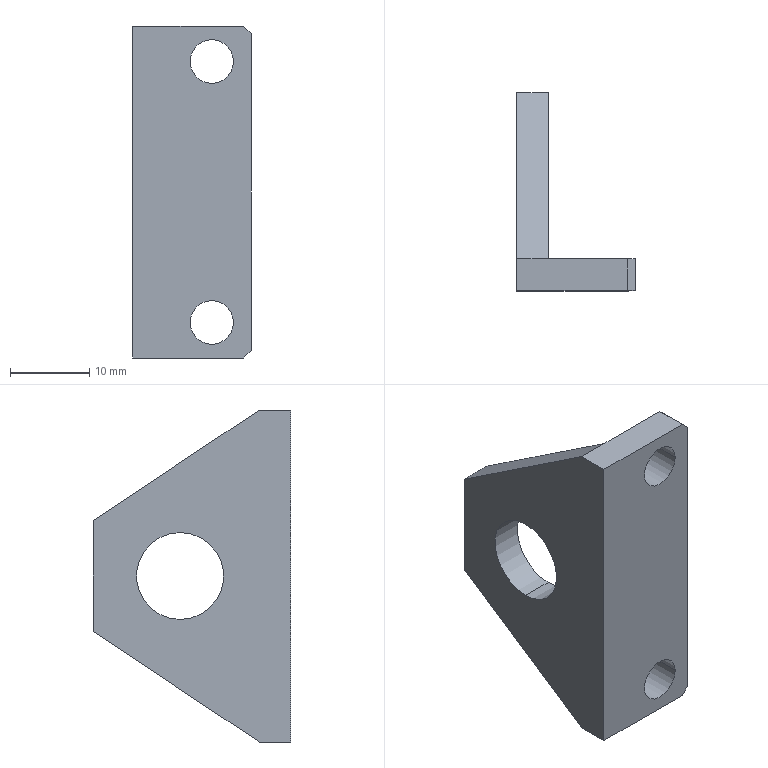Component | SolidWorks | 60100040019CylinderSupport-1 | 1 solid | 18 faces | box 15 x 25 x 42 mm | volume 4298 mm3 | plane 12 | cylinder 6 | commonest cylinder face diameters 5.5 x4 11 x2 | material Q235-A
build123d program:
from build123d import *

# Parameters (mm, degrees)
BOSS_EXTRUDE1_DEPTH = 4
SKETCH2_W           = 42
SKETCH2_H           = 4
BOSS_EXTRUDE2_DEPTH = 15
SKETCH3_R           = 5.5
CUT_EXTRUDE1_DEPTH  = 35.453
SKETCH4_R           = 2.75
CUT_EXTRUDE2_DEPTH  = 34.272
CHAMFER1_SIZE       = 1


with BuildPart() as part:
    # Sketch1 → Boss-Extrude1 (new body)
    with BuildSketch(Plane.XY):
        Polygon((-21, 0), (21, 0), (21, 4), (7, 25), (-7, 25), (-21, 4), align=None)
    extrude(amount=BOSS_EXTRUDE1_DEPTH)

    # Sketch2 → Boss-Extrude2 (add)
    with BuildSketch(Plane.XY):
        with Locations((0, 2)):
            Rectangle(SKETCH2_W, SKETCH2_H)
    extrude(amount=BOSS_EXTRUDE2_DEPTH)

    # Sketch3 → Cut-Extrude1 (cut, through all)
    with BuildSketch(Plane.XY.offset(4)):
        with Locations((0, 14)):
            Circle(SKETCH3_R)
    extrude(amount=-CUT_EXTRUDE1_DEPTH, mode=Mode.SUBTRACT)

    # Sketch4 → Cut-Extrude2 (cut, through all)
    with BuildSketch(Plane(origin=(0, 4, 0), x_dir=(1, 0, 0), z_dir=(0, 1, 0))):
        with Locations(Location((16.5, -10, 0), (0, 0, 270))):
            Circle(SKETCH4_R)
        with Locations(Location((-16.5, -10, 0), (0, 0, 270))):
            Circle(SKETCH4_R)
    extrude(amount=-CUT_EXTRUDE2_DEPTH, mode=Mode.SUBTRACT)

    # Chamfer1
    chamfer1_edges = [part.edges().sort_by_distance(p)[0] for p in [
        (-21, 2, 15),
        (21, 2, 15),
    ]]
    chamfer(chamfer1_edges, length=CHAMFER1_SIZE)


solid = part.part

# Placed as in the assembly
solid = solid.moved(Location((37.27, 8.768, 80.829), (0, 90, 0)))
STEP:
#1=COLOUR_RGB('',0.7922,0.8196,0.9333);
#2=FILL_AREA_STYLE_COLOUR('',#1);
#3=FILL_AREA_STYLE('',(#2));
#4=SURFACE_STYLE_FILL_AREA(#3);
#5=SURFACE_SIDE_STYLE('',(#4));
#6=SURFACE_STYLE_USAGE(.BOTH.,#5);
#7=PRESENTATION_STYLE_ASSIGNMENT((#6));
#8=CARTESIAN_POINT('',(1.753,0.3452,3.832));
#9=VERTEX_POINT('',#8);
#10=CARTESIAN_POINT('',(1.969,0.3452,3.832));
#11=VERTEX_POINT('',#10);
#12=CARTESIAN_POINT('',(1.861,0.3452,3.832));
#13=DIRECTION('',(0.,1.,0.));
#14=DIRECTION('',(1.,0.,0.));
#15=AXIS2_PLACEMENT_3D('',#12,#13,#14);
#16=CIRCLE('',#15,0.1083);
#17=EDGE_CURVE('',#9,#11,#16,.T.);
#18=ORIENTED_EDGE('',*,*,#17,.F.);
#19=CARTESIAN_POINT('',(1.753,0.5027,3.832));
#20=VERTEX_POINT('',#19);
#21=CARTESIAN_POINT('',(1.753,0.3452,3.832));
#22=DIRECTION('',(0.,1.,0.));
#23=VECTOR('',#22,39.37);
#24=LINE('',#21,#23);
#25=EDGE_CURVE('',#9,#20,#24,.T.);
#26=ORIENTED_EDGE('',*,*,#25,.T.);
#27=CARTESIAN_POINT('',(1.969,0.5027,3.832));
#28=VERTEX_POINT('',#27);
#29=CARTESIAN_POINT('',(1.861,0.5027,3.832));
#30=DIRECTION('',(0.,1.,0.));
#31=DIRECTION('',(1.,0.,0.));
#32=AXIS2_PLACEMENT_3D('',#29,#30,#31);
#33=CIRCLE('',#32,0.1083);
#34=EDGE_CURVE('',#20,#28,#33,.T.);
#35=ORIENTED_EDGE('',*,*,#34,.T.);
#36=CARTESIAN_POINT('',(1.969,0.3452,3.832));
#37=DIRECTION('',(0.,1.,0.));
#38=VECTOR('',#37,39.37);
#39=LINE('',#36,#38);
#40=EDGE_CURVE('',#11,#28,#39,.T.);
#41=ORIENTED_EDGE('',*,*,#40,.F.);
#42=EDGE_LOOP('',(#18,#26,#35,#41));
#43=FACE_OUTER_BOUND('',#42,.T.);
#44=CARTESIAN_POINT('',(1.861,0.3452,3.832));
#45=DIRECTION('',(0.,1.,0.));
#46=DIRECTION('',(1.,0.,0.));
#47=AXIS2_PLACEMENT_3D('',#44,#45,#46);
#48=CYLINDRICAL_SURFACE('',#47,0.1083);
#49=ADVANCED_FACE('',(#43),#48,.F.);
#50=CARTESIAN_POINT('',(1.753,0.3452,2.533));
#51=VERTEX_POINT('',#50);
#52=CARTESIAN_POINT('',(1.969,0.3452,2.533));
#53=VERTEX_POINT('',#52);
#54=CARTESIAN_POINT('',(1.861,0.3452,2.533));
#55=DIRECTION('',(0.,1.,0.));
#56=DIRECTION('',(1.,0.,0.));
#57=AXIS2_PLACEMENT_3D('',#54,#55,#56);
#58=CIRCLE('',#57,0.1083);
#59=EDGE_CURVE('',#51,#53,#58,.T.);
#60=ORIENTED_EDGE('',*,*,#59,.F.);
#61=CARTESIAN_POINT('',(1.753,0.5027,2.533));
#62=VERTEX_POINT('',#61);
#63=CARTESIAN_POINT('',(1.753,0.3452,2.533));
#64=DIRECTION('',(0.,1.,0.));
#65=VECTOR('',#64,39.37);
#66=LINE('',#63,#65);
#67=EDGE_CURVE('',#51,#62,#66,.T.);
#68=ORIENTED_EDGE('',*,*,#67,.T.);
#69=CARTESIAN_POINT('',(1.969,0.5027,2.533));
#70=VERTEX_POINT('',#69);
#71=CARTESIAN_POINT('',(1.861,0.5027,2.533));
#72=DIRECTION('',(0.,1.,0.));
#73=DIRECTION('',(1.,0.,0.));
#74=AXIS2_PLACEMENT_3D('',#71,#72,#73);
#75=CIRCLE('',#74,0.1083);
#76=EDGE_CURVE('',#62,#70,#75,.T.);
#77=ORIENTED_EDGE('',*,*,#76,.T.);
#78=CARTESIAN_POINT('',(1.969,0.3452,2.533));
#79=DIRECTION('',(0.,1.,0.));
#80=VECTOR('',#79,39.37);
#81=LINE('',#78,#80);
#82=EDGE_CURVE('',#53,#70,#81,.T.);
#83=ORIENTED_EDGE('',*,*,#82,.F.);
#84=EDGE_LOOP('',(#60,#68,#77,#83));
#85=FACE_OUTER_BOUND('',#84,.T.);
#86=CARTESIAN_POINT('',(1.861,0.3452,2.533));
#87=DIRECTION('',(0.,1.,0.));
#88=DIRECTION('',(1.,0.,0.));
#89=AXIS2_PLACEMENT_3D('',#86,#87,#88);
#90=CYLINDRICAL_SURFACE('',#89,0.1083);
#91=ADVANCED_FACE('',(#85),#90,.F.);
#92=CARTESIAN_POINT('',(1.467,0.8964,3.399));
#93=VERTEX_POINT('',#92);
#94=CARTESIAN_POINT('',(1.467,0.8964,2.966));
#95=VERTEX_POINT('',#94);
#96=CARTESIAN_POINT('',(1.467,0.8964,3.182));
#97=DIRECTION('',(1.,0.,0.));
#98=DIRECTION('',(0.,0.,-1.));
#99=AXIS2_PLACEMENT_3D('',#96,#97,#98);
#100=CIRCLE('',#99,0.2165);
#101=EDGE_CURVE('',#93,#95,#100,.T.);
#102=ORIENTED_EDGE('',*,*,#101,.F.);
#103=CARTESIAN_POINT('',(1.625,0.8964,3.399));
#104=VERTEX_POINT('',#103);
#105=CARTESIAN_POINT('',(1.467,0.8964,3.399));
#106=DIRECTION('',(1.,0.,0.));
#107=VECTOR('',#106,39.37);
#108=LINE('',#105,#107);
#109=EDGE_CURVE('',#93,#104,#108,.T.);
#110=ORIENTED_EDGE('',*,*,#109,.T.);
#111=CARTESIAN_POINT('',(1.625,0.8964,2.966));
#112=VERTEX_POINT('',#111);
#113=CARTESIAN_POINT('',(1.625,0.8964,3.182));
#114=DIRECTION('',(1.,0.,0.));
#115=DIRECTION('',(0.,0.,-1.));
#116=AXIS2_PLACEMENT_3D('',#113,#114,#115);
#117=CIRCLE('',#116,0.2165);
#118=EDGE_CURVE('',#104,#112,#117,.T.);
#119=ORIENTED_EDGE('',*,*,#118,.T.);
#120=CARTESIAN_POINT('',(1.467,0.8964,2.966));
#121=DIRECTION('',(1.,0.,0.));
#122=VECTOR('',#121,39.37);
#123=LINE('',#120,#122);
#124=EDGE_CURVE('',#95,#112,#123,.T.);
#125=ORIENTED_EDGE('',*,*,#124,.F.);
#126=EDGE_LOOP('',(#102,#110,#119,#125));
#127=FACE_OUTER_BOUND('',#126,.T.);
#128=CARTESIAN_POINT('',(1.467,0.8964,3.182));
#129=DIRECTION('',(1.,0.,0.));
#130=DIRECTION('',(0.,0.,-1.));
#131=AXIS2_PLACEMENT_3D('',#128,#129,#130);
#132=CYLINDRICAL_SURFACE('',#131,0.2165);
#133=ADVANCED_FACE('',(#127),#132,.F.);
#134=CARTESIAN_POINT('',(1.625,0.8964,3.182));
#135=DIRECTION('',(1.,0.,0.));
#136=DIRECTION('',(0.,0.,-1.));
#137=AXIS2_PLACEMENT_3D('',#134,#135,#136);
#138=CIRCLE('',#137,0.2165);
#139=EDGE_CURVE('',#112,#104,#138,.T.);
#140=ORIENTED_EDGE('',*,*,#139,.F.);
#141=ORIENTED_EDGE('',*,*,#118,.F.);
#142=EDGE_LOOP('',(#140,#141));
#143=FACE_BOUND('',#142,.T.);
#144=CARTESIAN_POINT('',(1.625,1.329,3.458));
#145=VERTEX_POINT('',#144);
#146=CARTESIAN_POINT('',(1.625,0.5027,4.009));
#147=VERTEX_POINT('',#146);
#148=CARTESIAN_POINT('',(1.625,1.329,3.458));
#149=DIRECTION('',(0.,-0.8321,0.5547));
#150=VECTOR('',#149,39.37);
#151=LINE('',#148,#150);
#152=EDGE_CURVE('',#145,#147,#151,.T.);
#153=ORIENTED_EDGE('',*,*,#152,.T.);
#154=CARTESIAN_POINT('',(1.625,0.5027,2.355));
#155=VERTEX_POINT('',#154);
#156=CARTESIAN_POINT('',(1.625,0.5027,4.009));
#157=DIRECTION('',(0.,0.,-1.));
#158=VECTOR('',#157,39.37);
#159=LINE('',#156,#158);
#160=EDGE_CURVE('',#147,#155,#159,.T.);
#161=ORIENTED_EDGE('',*,*,#160,.T.);
#162=CARTESIAN_POINT('',(1.625,1.329,2.907));
#163=VERTEX_POINT('',#162);
#164=CARTESIAN_POINT('',(1.625,1.329,2.907));
#165=DIRECTION('',(0.,0.8321,0.5547));
#166=VECTOR('',#165,39.37);
#167=LINE('',#164,#166);
#168=EDGE_CURVE('',#155,#163,#167,.T.);
#169=ORIENTED_EDGE('',*,*,#168,.T.);
#170=CARTESIAN_POINT('',(1.625,1.329,2.907));
#171=DIRECTION('',(0.,0.,1.));
#172=VECTOR('',#171,39.37);
#173=LINE('',#170,#172);
#174=EDGE_CURVE('',#163,#145,#173,.T.);
#175=ORIENTED_EDGE('',*,*,#174,.T.);
#176=EDGE_LOOP('',(#153,#161,#169,#175));
#177=FACE_OUTER_BOUND('',#176,.T.);
#178=CARTESIAN_POINT('',(1.625,0.3452,4.009));
#179=DIRECTION('',(1.,0.,0.));
#180=DIRECTION('',(0.,0.,-1.));
#181=AXIS2_PLACEMENT_3D('',#178,#179,#180);
#182=PLANE('',#181);
#183=ADVANCED_FACE('',(#143,#177),#182,.T.);
#184=CARTESIAN_POINT('',(2.019,0.3452,4.009));
#185=VERTEX_POINT('',#184);
#186=CARTESIAN_POINT('',(1.467,0.3452,4.009));
#187=VERTEX_POINT('',#186);
#188=CARTESIAN_POINT('',(1.625,0.3452,4.009));
#189=DIRECTION('',(-1.,0.,0.));
#190=VECTOR('',#189,39.37);
#191=LINE('',#188,#190);
#192=EDGE_CURVE('',#185,#187,#191,.T.);
#193=ORIENTED_EDGE('',*,*,#192,.F.);
#194=CARTESIAN_POINT('',(2.019,0.5027,4.009));
#195=VERTEX_POINT('',#194);
#196=CARTESIAN_POINT('',(2.019,0.5027,4.009));
#197=DIRECTION('',(0.,1.,0.));
#198=VECTOR('',#197,39.37);
#199=LINE('',#196,#198);
#200=EDGE_CURVE('',#185,#195,#199,.T.);
#201=ORIENTED_EDGE('',*,*,#200,.T.);
#202=CARTESIAN_POINT('',(2.058,0.5027,4.009));
#203=DIRECTION('',(-1.,0.,0.));
#204=VECTOR('',#203,39.37);
#205=LINE('',#202,#204);
#206=EDGE_CURVE('',#195,#147,#205,.T.);
#207=ORIENTED_EDGE('',*,*,#206,.T.);
#208=CARTESIAN_POINT('',(1.467,0.5027,4.009));
#209=VERTEX_POINT('',#208);
#210=CARTESIAN_POINT('',(1.625,0.5027,4.009));
#211=DIRECTION('',(-1.,0.,0.));
#212=VECTOR('',#211,39.37);
#213=LINE('',#210,#212);
#214=EDGE_CURVE('',#147,#209,#213,.T.);
#215=ORIENTED_EDGE('',*,*,#214,.T.);
#216=CARTESIAN_POINT('',(1.467,0.5027,4.009));
#217=DIRECTION('',(0.,-1.,0.));
#218=VECTOR('',#217,39.37);
#219=LINE('',#216,#218);
#220=EDGE_CURVE('',#209,#187,#219,.T.);
#221=ORIENTED_EDGE('',*,*,#220,.T.);
#222=EDGE_LOOP('',(#193,#201,#207,#215,#221));
#223=FACE_OUTER_BOUND('',#222,.T.);
#224=CARTESIAN_POINT('',(1.625,0.5027,4.009));
#225=DIRECTION('',(0.,0.,-1.));
#226=DIRECTION('',(-1.,0.,0.));
#227=AXIS2_PLACEMENT_3D('',#224,#225,#226);
#228=PLANE('',#227);
#229=ADVANCED_FACE('',(#223),#228,.F.);
#230=CARTESIAN_POINT('',(1.861,0.3452,3.832));
#231=DIRECTION('',(0.,1.,0.));
#232=DIRECTION('',(1.,0.,0.));
#233=AXIS2_PLACEMENT_3D('',#230,#231,#232);
#234=CIRCLE('',#233,0.1083);
#235=EDGE_CURVE('',#11,#9,#234,.T.);
#236=ORIENTED_EDGE('',*,*,#235,.T.);
#237=ORIENTED_EDGE('',*,*,#17,.T.);
#238=EDGE_LOOP('',(#236,#237));
#239=FACE_BOUND('',#238,.T.);
#240=CARTESIAN_POINT('',(1.861,0.3452,2.533));
#241=DIRECTION('',(0.,1.,0.));
#242=DIRECTION('',(1.,0.,0.));
#243=AXIS2_PLACEMENT_3D('',#240,#241,#242);
#244=CIRCLE('',#243,0.1083);
#245=EDGE_CURVE('',#53,#51,#244,.T.);
#246=ORIENTED_EDGE('',*,*,#245,.T.);
#247=ORIENTED_EDGE('',*,*,#59,.T.);
#248=EDGE_LOOP('',(#246,#247));
#249=FACE_BOUND('',#248,.T.);
#250=CARTESIAN_POINT('',(2.019,0.3452,2.355));
#251=VERTEX_POINT('',#250);
#252=CARTESIAN_POINT('',(1.467,0.3452,2.355));
#253=VERTEX_POINT('',#252);
#254=CARTESIAN_POINT('',(1.625,0.3452,2.355));
#255=DIRECTION('',(-1.,0.,0.));
#256=VECTOR('',#255,39.37);
#257=LINE('',#254,#256);
#258=EDGE_CURVE('',#251,#253,#257,.T.);
#259=ORIENTED_EDGE('',*,*,#258,.F.);
#260=CARTESIAN_POINT('',(2.058,0.3452,2.395));
#261=VERTEX_POINT('',#260);
#262=CARTESIAN_POINT('',(2.058,0.3452,2.395));
#263=DIRECTION('',(0.7071,0.,0.7071));
#264=VECTOR('',#263,39.37);
#265=LINE('',#262,#264);
#266=EDGE_CURVE('',#251,#261,#265,.T.);
#267=ORIENTED_EDGE('',*,*,#266,.T.);
#268=CARTESIAN_POINT('',(2.058,0.3452,3.97));
#269=VERTEX_POINT('',#268);
#270=CARTESIAN_POINT('',(2.058,0.3452,4.009));
#271=DIRECTION('',(0.,0.,-1.));
#272=VECTOR('',#271,39.37);
#273=LINE('',#270,#272);
#274=EDGE_CURVE('',#269,#261,#273,.T.);
#275=ORIENTED_EDGE('',*,*,#274,.F.);
#276=CARTESIAN_POINT('',(2.058,0.3452,3.97));
#277=DIRECTION('',(-0.7071,0.,0.7071));
#278=VECTOR('',#277,39.37);
#279=LINE('',#276,#278);
#280=EDGE_CURVE('',#269,#185,#279,.T.);
#281=ORIENTED_EDGE('',*,*,#280,.T.);
#282=ORIENTED_EDGE('',*,*,#192,.T.);
#283=CARTESIAN_POINT('',(1.467,0.3452,4.009));
#284=DIRECTION('',(0.,0.,-1.));
#285=VECTOR('',#284,39.37);
#286=LINE('',#283,#285);
#287=EDGE_CURVE('',#187,#253,#286,.T.);
#288=ORIENTED_EDGE('',*,*,#287,.T.);
#289=EDGE_LOOP('',(#259,#267,#275,#281,#282,#288));
#290=FACE_OUTER_BOUND('',#289,.T.);
#291=CARTESIAN_POINT('',(1.625,0.3452,4.009));
#292=DIRECTION('',(0.,1.,0.));
#293=DIRECTION('',(1.,0.,0.));
#294=AXIS2_PLACEMENT_3D('',#291,#292,#293);
#295=PLANE('',#294);
#296=ADVANCED_FACE('',(#239,#249,#290),#295,.F.);
#297=CARTESIAN_POINT('',(2.019,0.5027,2.355));
#298=VERTEX_POINT('',#297);
#299=CARTESIAN_POINT('',(2.058,0.5027,2.355));
#300=DIRECTION('',(-1.,0.,0.));
#301=VECTOR('',#300,39.37);
#302=LINE('',#299,#301);
#303=EDGE_CURVE('',#298,#155,#302,.T.);
#304=ORIENTED_EDGE('',*,*,#303,.F.);
#305=CARTESIAN_POINT('',(2.019,0.5027,2.355));
#306=DIRECTION('',(0.,-1.,0.));
#307=VECTOR('',#306,39.37);
#308=LINE('',#305,#307);
#309=EDGE_CURVE('',#298,#251,#308,.T.);
#310=ORIENTED_EDGE('',*,*,#309,.T.);
#311=ORIENTED_EDGE('',*,*,#258,.T.);
#312=CARTESIAN_POINT('',(1.467,0.5027,2.355));
#313=VERTEX_POINT('',#312);
#314=CARTESIAN_POINT('',(1.467,0.5027,2.355));
#315=DIRECTION('',(0.,1.,0.));
#316=VECTOR('',#315,39.37);
#317=LINE('',#314,#316);
#318=EDGE_CURVE('',#253,#313,#317,.T.);
#319=ORIENTED_EDGE('',*,*,#318,.T.);
#320=CARTESIAN_POINT('',(1.625,0.5027,2.355));
#321=DIRECTION('',(-1.,0.,0.));
#322=VECTOR('',#321,39.37);
#323=LINE('',#320,#322);
#324=EDGE_CURVE('',#155,#313,#323,.T.);
#325=ORIENTED_EDGE('',*,*,#324,.F.);
#326=EDGE_LOOP('',(#304,#310,#311,#319,#325));
#327=FACE_OUTER_BOUND('',#326,.T.);
#328=CARTESIAN_POINT('',(1.625,0.5027,2.355));
#329=DIRECTION('',(0.,0.,1.));
#330=DIRECTION('',(1.,0.,0.));
#331=AXIS2_PLACEMENT_3D('',#328,#329,#330);
#332=PLANE('',#331);
#333=ADVANCED_FACE('',(#327),#332,.F.);
#334=CARTESIAN_POINT('',(1.467,1.329,2.907));
#335=VERTEX_POINT('',#334);
#336=CARTESIAN_POINT('',(1.467,1.329,2.907));
#337=DIRECTION('',(0.,0.8321,0.5547));
#338=VECTOR('',#337,39.37);
#339=LINE('',#336,#338);
#340=EDGE_CURVE('',#313,#335,#339,.T.);
#341=ORIENTED_EDGE('',*,*,#340,.T.);
#342=CARTESIAN_POINT('',(1.625,1.329,2.907));
#343=DIRECTION('',(-1.,0.,0.));
#344=VECTOR('',#343,39.37);
#345=LINE('',#342,#344);
#346=EDGE_CURVE('',#163,#335,#345,.T.);
#347=ORIENTED_EDGE('',*,*,#346,.F.);
#348=ORIENTED_EDGE('',*,*,#168,.F.);
#349=ORIENTED_EDGE('',*,*,#324,.T.);
#350=EDGE_LOOP('',(#341,#347,#348,#349));
#351=FACE_OUTER_BOUND('',#350,.T.);
#352=CARTESIAN_POINT('',(1.625,1.329,2.907));
#353=DIRECTION('',(0.,-0.5547,0.8321));
#354=DIRECTION('',(0.,-0.8321,-0.5547));
#355=AXIS2_PLACEMENT_3D('',#352,#353,#354);
#356=PLANE('',#355);
#357=ADVANCED_FACE('',(#351),#356,.F.);
#358=CARTESIAN_POINT('',(1.467,1.329,3.458));
#359=VERTEX_POINT('',#358);
#360=CARTESIAN_POINT('',(1.467,1.329,2.907));
#361=DIRECTION('',(0.,0.,1.));
#362=VECTOR('',#361,39.37);
#363=LINE('',#360,#362);
#364=EDGE_CURVE('',#335,#359,#363,.T.);
#365=ORIENTED_EDGE('',*,*,#364,.T.);
#366=CARTESIAN_POINT('',(1.625,1.329,3.458));
#367=DIRECTION('',(-1.,0.,0.));
#368=VECTOR('',#367,39.37);
#369=LINE('',#366,#368);
#370=EDGE_CURVE('',#145,#359,#369,.T.);
#371=ORIENTED_EDGE('',*,*,#370,.F.);
#372=ORIENTED_EDGE('',*,*,#174,.F.);
#373=ORIENTED_EDGE('',*,*,#346,.T.);
#374=EDGE_LOOP('',(#365,#371,#372,#373));
#375=FACE_OUTER_BOUND('',#374,.T.);
#376=CARTESIAN_POINT('',(1.625,1.329,2.907));
#377=DIRECTION('',(0.,-1.,0.));
#378=DIRECTION('',(-1.,0.,0.));
#379=AXIS2_PLACEMENT_3D('',#376,#377,#378);
#380=PLANE('',#379);
#381=ADVANCED_FACE('',(#375),#380,.F.);
#382=CARTESIAN_POINT('',(1.467,1.329,3.458));
#383=DIRECTION('',(0.,-0.8321,0.5547));
#384=VECTOR('',#383,39.37);
#385=LINE('',#382,#384);
#386=EDGE_CURVE('',#359,#209,#385,.T.);
#387=ORIENTED_EDGE('',*,*,#386,.T.);
#388=ORIENTED_EDGE('',*,*,#214,.F.);
#389=ORIENTED_EDGE('',*,*,#152,.F.);
#390=ORIENTED_EDGE('',*,*,#370,.T.);
#391=EDGE_LOOP('',(#387,#388,#389,#390));
#392=FACE_OUTER_BOUND('',#391,.T.);
#393=CARTESIAN_POINT('',(1.625,1.329,3.458));
#394=DIRECTION('',(0.,-0.5547,-0.8321));
#395=DIRECTION('',(0.,0.8321,-0.5547));
#396=AXIS2_PLACEMENT_3D('',#393,#394,#395);
#397=PLANE('',#396);
#398=ADVANCED_FACE('',(#392),#397,.F.);
#399=CARTESIAN_POINT('',(1.467,0.8964,3.182));
#400=DIRECTION('',(1.,0.,0.));
#401=DIRECTION('',(0.,0.,-1.));
#402=AXIS2_PLACEMENT_3D('',#399,#400,#401);
#403=CIRCLE('',#402,0.2165);
#404=EDGE_CURVE('',#95,#93,#403,.T.);
#405=ORIENTED_EDGE('',*,*,#404,.T.);
#406=ORIENTED_EDGE('',*,*,#101,.T.);
#407=EDGE_LOOP('',(#405,#406));
#408=FACE_BOUND('',#407,.T.);
#409=ORIENTED_EDGE('',*,*,#220,.F.);
#410=ORIENTED_EDGE('',*,*,#386,.F.);
#411=ORIENTED_EDGE('',*,*,#364,.F.);
#412=ORIENTED_EDGE('',*,*,#340,.F.);
#413=ORIENTED_EDGE('',*,*,#318,.F.);
#414=ORIENTED_EDGE('',*,*,#287,.F.);
#415=EDGE_LOOP('',(#409,#410,#411,#412,#413,#414));
#416=FACE_OUTER_BOUND('',#415,.T.);
#417=CARTESIAN_POINT('',(1.467,0.3452,4.009));
#418=DIRECTION('',(1.,0.,0.));
#419=DIRECTION('',(0.,0.,-1.));
#420=AXIS2_PLACEMENT_3D('',#417,#418,#419);
#421=PLANE('',#420);
#422=ADVANCED_FACE('',(#408,#416),#421,.F.);
#423=CARTESIAN_POINT('',(1.861,0.5027,3.832));
#424=DIRECTION('',(0.,1.,0.));
#425=DIRECTION('',(1.,0.,0.));
#426=AXIS2_PLACEMENT_3D('',#423,#424,#425);
#427=CIRCLE('',#426,0.1083);
#428=EDGE_CURVE('',#28,#20,#427,.T.);
#429=ORIENTED_EDGE('',*,*,#428,.F.);
#430=ORIENTED_EDGE('',*,*,#34,.F.);
#431=EDGE_LOOP('',(#429,#430));
#432=FACE_BOUND('',#431,.T.);
#433=CARTESIAN_POINT('',(1.861,0.5027,2.533));
#434=DIRECTION('',(0.,1.,0.));
#435=DIRECTION('',(1.,0.,0.));
#436=AXIS2_PLACEMENT_3D('',#433,#434,#435);
#437=CIRCLE('',#436,0.1083);
#438=EDGE_CURVE('',#70,#62,#437,.T.);
#439=ORIENTED_EDGE('',*,*,#438,.F.);
#440=ORIENTED_EDGE('',*,*,#76,.F.);
#441=EDGE_LOOP('',(#439,#440));
#442=FACE_BOUND('',#441,.T.);
#443=CARTESIAN_POINT('',(2.058,0.5027,2.395));
#444=VERTEX_POINT('',#443);
#445=CARTESIAN_POINT('',(2.058,0.5027,3.97));
#446=VERTEX_POINT('',#445);
#447=CARTESIAN_POINT('',(2.058,0.5027,4.009));
#448=DIRECTION('',(0.,0.,1.));
#449=VECTOR('',#448,39.37);
#450=LINE('',#447,#449);
#451=EDGE_CURVE('',#444,#446,#450,.T.);
#452=ORIENTED_EDGE('',*,*,#451,.F.);
#453=CARTESIAN_POINT('',(2.058,0.5027,2.395));
#454=DIRECTION('',(-0.7071,0.,-0.7071));
#455=VECTOR('',#454,39.37);
#456=LINE('',#453,#455);
#457=EDGE_CURVE('',#444,#298,#456,.T.);
#458=ORIENTED_EDGE('',*,*,#457,.T.);
#459=ORIENTED_EDGE('',*,*,#303,.T.);
#460=ORIENTED_EDGE('',*,*,#160,.F.);
#461=ORIENTED_EDGE('',*,*,#206,.F.);
#462=CARTESIAN_POINT('',(2.058,0.5027,3.97));
#463=DIRECTION('',(0.7071,0.,-0.7071));
#464=VECTOR('',#463,39.37);
#465=LINE('',#462,#464);
#466=EDGE_CURVE('',#195,#446,#465,.T.);
#467=ORIENTED_EDGE('',*,*,#466,.T.);
#468=EDGE_LOOP('',(#452,#458,#459,#460,#461,#467));
#469=FACE_OUTER_BOUND('',#468,.T.);
#470=CARTESIAN_POINT('',(2.058,0.5027,4.009));
#471=DIRECTION('',(0.,-1.,0.));
#472=DIRECTION('',(-1.,0.,0.));
#473=AXIS2_PLACEMENT_3D('',#470,#471,#472);
#474=PLANE('',#473);
#475=ADVANCED_FACE('',(#432,#442,#469),#474,.F.);
#476=ORIENTED_EDGE('',*,*,#274,.T.);
#477=CARTESIAN_POINT('',(2.058,0.5027,2.395));
#478=DIRECTION('',(0.,1.,0.));
#479=VECTOR('',#478,39.37);
#480=LINE('',#477,#479);
#481=EDGE_CURVE('',#261,#444,#480,.T.);
#482=ORIENTED_EDGE('',*,*,#481,.T.);
#483=ORIENTED_EDGE('',*,*,#451,.T.);
#484=CARTESIAN_POINT('',(2.058,0.5027,3.97));
#485=DIRECTION('',(0.,-1.,0.));
#486=VECTOR('',#485,39.37);
#487=LINE('',#484,#486);
#488=EDGE_CURVE('',#446,#269,#487,.T.);
#489=ORIENTED_EDGE('',*,*,#488,.T.);
#490=EDGE_LOOP('',(#476,#482,#483,#489));
#491=FACE_OUTER_BOUND('',#490,.T.);
#492=CARTESIAN_POINT('',(2.058,0.5027,4.009));
#493=DIRECTION('',(-1.,0.,0.));
#494=DIRECTION('',(0.,0.,1.));
#495=AXIS2_PLACEMENT_3D('',#492,#493,#494);
#496=PLANE('',#495);
#497=ADVANCED_FACE('',(#491),#496,.F.);
#498=ORIENTED_EDGE('',*,*,#109,.F.);
#499=ORIENTED_EDGE('',*,*,#404,.F.);
#500=ORIENTED_EDGE('',*,*,#124,.T.);
#501=ORIENTED_EDGE('',*,*,#139,.T.);
#502=EDGE_LOOP('',(#498,#499,#500,#501));
#503=FACE_OUTER_BOUND('',#502,.T.);
#504=CARTESIAN_POINT('',(1.467,0.8964,3.182));
#505=DIRECTION('',(1.,0.,0.));
#506=DIRECTION('',(0.,0.,-1.));
#507=AXIS2_PLACEMENT_3D('',#504,#505,#506);
#508=CYLINDRICAL_SURFACE('',#507,0.2165);
#509=ADVANCED_FACE('',(#503),#508,.F.);
#510=ORIENTED_EDGE('',*,*,#67,.F.);
#511=ORIENTED_EDGE('',*,*,#245,.F.);
#512=ORIENTED_EDGE('',*,*,#82,.T.);
#513=ORIENTED_EDGE('',*,*,#438,.T.);
#514=EDGE_LOOP('',(#510,#511,#512,#513));
#515=FACE_OUTER_BOUND('',#514,.T.);
#516=CARTESIAN_POINT('',(1.861,0.3452,2.533));
#517=DIRECTION('',(0.,1.,0.));
#518=DIRECTION('',(1.,0.,0.));
#519=AXIS2_PLACEMENT_3D('',#516,#517,#518);
#520=CYLINDRICAL_SURFACE('',#519,0.1083);
#521=ADVANCED_FACE('',(#515),#520,.F.);
#522=ORIENTED_EDGE('',*,*,#25,.F.);
#523=ORIENTED_EDGE('',*,*,#235,.F.);
#524=ORIENTED_EDGE('',*,*,#40,.T.);
#525=ORIENTED_EDGE('',*,*,#428,.T.);
#526=EDGE_LOOP('',(#522,#523,#524,#525));
#527=FACE_OUTER_BOUND('',#526,.T.);
#528=CARTESIAN_POINT('',(1.861,0.3452,3.832));
#529=DIRECTION('',(0.,1.,0.));
#530=DIRECTION('',(1.,0.,0.));
#531=AXIS2_PLACEMENT_3D('',#528,#529,#530);
#532=CYLINDRICAL_SURFACE('',#531,0.1083);
#533=ADVANCED_FACE('',(#527),#532,.F.);
#534=ORIENTED_EDGE('',*,*,#266,.F.);
#535=ORIENTED_EDGE('',*,*,#309,.F.);
#536=ORIENTED_EDGE('',*,*,#457,.F.);
#537=ORIENTED_EDGE('',*,*,#481,.F.);
#538=EDGE_LOOP('',(#534,#535,#536,#537));
#539=FACE_OUTER_BOUND('',#538,.T.);
#540=CARTESIAN_POINT('',(2.058,0.5027,2.395));
#541=DIRECTION('',(-0.7071,0.,0.7071));
#542=DIRECTION('',(0.7071,0.,0.7071));
#543=AXIS2_PLACEMENT_3D('',#540,#541,#542);
#544=PLANE('',#543);
#545=ADVANCED_FACE('',(#539),#544,.F.);
#546=ORIENTED_EDGE('',*,*,#466,.F.);
#547=ORIENTED_EDGE('',*,*,#200,.F.);
#548=ORIENTED_EDGE('',*,*,#280,.F.);
#549=ORIENTED_EDGE('',*,*,#488,.F.);
#550=EDGE_LOOP('',(#546,#547,#548,#549));
#551=FACE_OUTER_BOUND('',#550,.T.);
#552=CARTESIAN_POINT('',(2.058,0.5027,3.97));
#553=DIRECTION('',(-0.7071,0.,-0.7071));
#554=DIRECTION('',(-0.7071,0.,0.7071));
#555=AXIS2_PLACEMENT_3D('',#552,#553,#554);
#556=PLANE('',#555);
#557=ADVANCED_FACE('',(#551),#556,.F.);
#558=CLOSED_SHELL('',(#49,#91,#133,#183,#229,#296,#333,#357,#381,#398,#422,#475,#497,#509,#521,#533,#545,#557));
#559=MANIFOLD_SOLID_BREP('',#558);
#560=STYLED_ITEM('',(#7),#559);
#561=(LENGTH_UNIT()NAMED_UNIT(*)SI_UNIT($,.METRE.));
#562=LENGTH_MEASURE_WITH_UNIT(LENGTH_MEASURE(0.0254),#561);
#563=DIMENSIONAL_EXPONENTS(1.,0.,0.,0.,0.,0.,0.);
#564=(CONVERSION_BASED_UNIT('',#562)LENGTH_UNIT()NAMED_UNIT(#563));
#565=UNCERTAINTY_MEASURE_WITH_UNIT(LENGTH_MEASURE(0.00001),#564,'','');
#566=(NAMED_UNIT(*)PLANE_ANGLE_UNIT()SI_UNIT($,.RADIAN.));
#567=(NAMED_UNIT(*)SI_UNIT($,.STERADIAN.)SOLID_ANGLE_UNIT());
#568=(GEOMETRIC_REPRESENTATION_CONTEXT(3)GLOBAL_UNCERTAINTY_ASSIGNED_CONTEXT((#565))GLOBAL_UNIT_ASSIGNED_CONTEXT((#564,#566,#567))REPRESENTATION_CONTEXT('',''));
#569=MECHANICAL_DESIGN_GEOMETRIC_PRESENTATION_REPRESENTATION('',(#560),#568);
#570=CARTESIAN_POINT('',(0.,0.,0.));
#571=DIRECTION('',(0.,0.,1.));
#572=DIRECTION('',(1.,0.,0.));
#573=AXIS2_PLACEMENT_3D('',#570,#571,#572);
#574=(LENGTH_UNIT()NAMED_UNIT(*)SI_UNIT($,.METRE.));
#575=LENGTH_MEASURE_WITH_UNIT(LENGTH_MEASURE(0.0254),#574);
#576=DIMENSIONAL_EXPONENTS(1.,0.,0.,0.,0.,0.,0.);
#577=(CONVERSION_BASED_UNIT('',#575)LENGTH_UNIT()NAMED_UNIT(#576));
#578=UNCERTAINTY_MEASURE_WITH_UNIT(LENGTH_MEASURE(0.00001),#577,'','');
#579=(NAMED_UNIT(*)PLANE_ANGLE_UNIT()SI_UNIT($,.RADIAN.));
#580=(NAMED_UNIT(*)SI_UNIT($,.STERADIAN.)SOLID_ANGLE_UNIT());
#581=(GEOMETRIC_REPRESENTATION_CONTEXT(3)GLOBAL_UNCERTAINTY_ASSIGNED_CONTEXT((#578))GLOBAL_UNIT_ASSIGNED_CONTEXT((#577,#579,#580))REPRESENTATION_CONTEXT('',''));
#582=ADVANCED_BREP_SHAPE_REPRESENTATION('',(#559,#573),#581);
#583=PRESENTATION_LAYER_ASSIGNMENT('','',(#560));